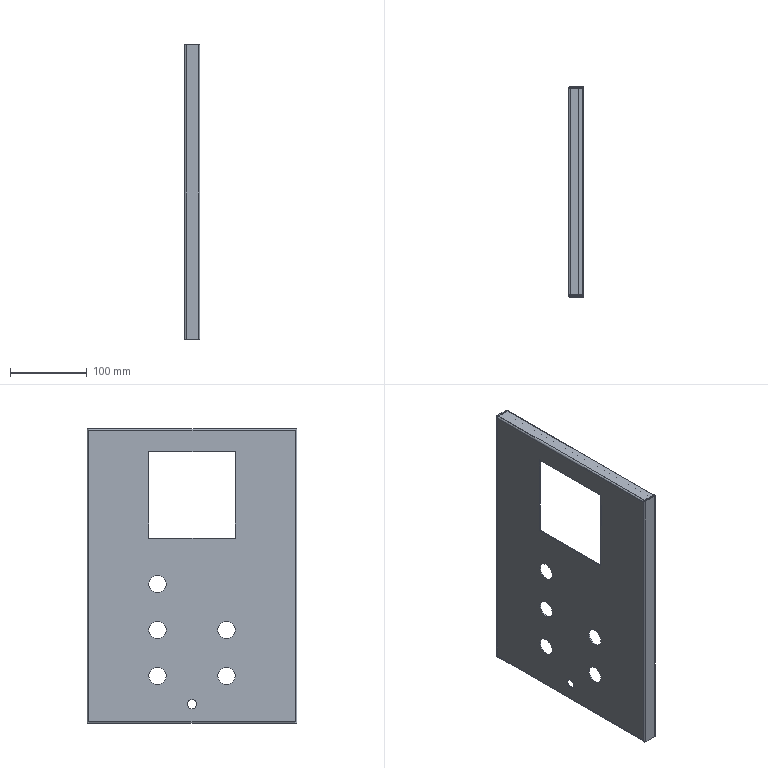Component | SolidWorks | CompensationInnerDoorAssembly100-2_CompensationChamberDoorPanel-1 | 1 solid | 90 faces | volume 147320 mm3 | plane 62 | cylinder 28 | commonest cylinder face diameters 22.5 x10 4.8 x4 2.4 x4 2.5 x4 0.1 x4 12 x2